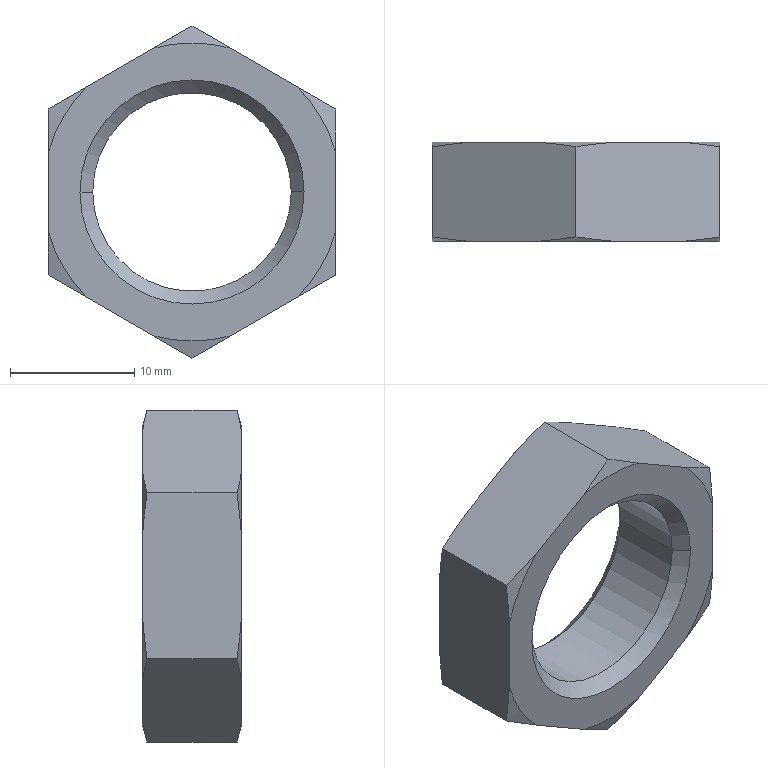Component | SolidWorks | GB_T6172.1-2000HexThinNutAAndBM16-3 | 1 solid | 26 faces | box 23.17 x 8 x 26.75 mm | volume 2049 mm3 | cone 16 | plane 8 | cylinder 2 | commonest cylinder face diameters 16 x2 | material 04 Grade
STEP:
#1=CARTESIAN_POINT('',(-12.126,-0.5893,-13.85));
#2=VERTEX_POINT('',#1);
#3=CARTESIAN_POINT('',(-11.496,-0.5893,-13.847));
#4=VERTEX_POINT('',#3);
#5=CARTESIAN_POINT('',(-11.811,-0.5893,-13.848));
#6=DIRECTION('',(0.,-1.,-0.));
#7=DIRECTION('',(-1.,0.,-0.003934));
#8=AXIS2_PLACEMENT_3D('',#5,#6,#7);
#9=CIRCLE('',#8,0.315);
#10=EDGE_CURVE('',#2,#4,#9,.T.);
#11=ORIENTED_EDGE('',*,*,#10,.F.);
#12=CARTESIAN_POINT('',(-12.167,-0.6299,-13.85));
#13=VERTEX_POINT('',#12);
#14=CARTESIAN_POINT('',(-12.126,-0.5893,-13.85));
#15=DIRECTION('',(-0.7071,-0.7071,-0.002781));
#16=VECTOR('',#15,39.37);
#17=LINE('',#14,#16);
#18=EDGE_CURVE('',#2,#13,#17,.T.);
#19=ORIENTED_EDGE('',*,*,#18,.T.);
#20=CARTESIAN_POINT('',(-11.455,-0.6299,-13.847));
#21=VERTEX_POINT('',#20);
#22=CARTESIAN_POINT('',(-11.811,-0.6299,-13.848));
#23=DIRECTION('',(-0.,1.,0.));
#24=DIRECTION('',(-1.,0.,-0.003934));
#25=AXIS2_PLACEMENT_3D('',#22,#23,#24);
#26=CIRCLE('',#25,0.3555);
#27=EDGE_CURVE('',#21,#13,#26,.T.);
#28=ORIENTED_EDGE('',*,*,#27,.F.);
#29=CARTESIAN_POINT('',(-11.496,-0.5893,-13.847));
#30=DIRECTION('',(0.7071,-0.7071,0.002781));
#31=VECTOR('',#30,39.37);
#32=LINE('',#29,#31);
#33=EDGE_CURVE('',#4,#21,#32,.T.);
#34=ORIENTED_EDGE('',*,*,#33,.F.);
#35=EDGE_LOOP('',(#11,#19,#28,#34));
#36=FACE_OUTER_BOUND('',#35,.T.);
#37=CARTESIAN_POINT('',(-11.811,-0.5893,-13.848));
#38=DIRECTION('',(0.,-1.,-0.));
#39=DIRECTION('',(1.,0.,0.003934));
#40=AXIS2_PLACEMENT_3D('',#37,#38,#39);
#41=CONICAL_SURFACE('',#40,0.315,0.7854);
#42=ADVANCED_FACE('',(#36),#41,.F.);
#43=CARTESIAN_POINT('',(-11.496,-0.3555,-13.847));
#44=VERTEX_POINT('',#43);
#45=CARTESIAN_POINT('',(-12.126,-0.3555,-13.85));
#46=VERTEX_POINT('',#45);
#47=CARTESIAN_POINT('',(-11.811,-0.3555,-13.848));
#48=DIRECTION('',(-0.,1.,0.));
#49=DIRECTION('',(-1.,0.,-0.003934));
#50=AXIS2_PLACEMENT_3D('',#47,#48,#49);
#51=CIRCLE('',#50,0.315);
#52=EDGE_CURVE('',#44,#46,#51,.T.);
#53=ORIENTED_EDGE('',*,*,#52,.F.);
#54=CARTESIAN_POINT('',(-11.455,-0.315,-13.847));
#55=VERTEX_POINT('',#54);
#56=CARTESIAN_POINT('',(-11.455,-0.315,-13.847));
#57=DIRECTION('',(0.7071,0.7071,0.002781));
#58=VECTOR('',#57,39.37);
#59=LINE('',#56,#58);
#60=EDGE_CURVE('',#44,#55,#59,.T.);
#61=ORIENTED_EDGE('',*,*,#60,.T.);
#62=CARTESIAN_POINT('',(-12.167,-0.315,-13.85));
#63=VERTEX_POINT('',#62);
#64=CARTESIAN_POINT('',(-11.811,-0.315,-13.848));
#65=DIRECTION('',(0.,-1.,-0.));
#66=DIRECTION('',(-1.,0.,-0.003934));
#67=AXIS2_PLACEMENT_3D('',#64,#65,#66);
#68=CIRCLE('',#67,0.3555);
#69=EDGE_CURVE('',#63,#55,#68,.T.);
#70=ORIENTED_EDGE('',*,*,#69,.F.);
#71=CARTESIAN_POINT('',(-12.167,-0.315,-13.85));
#72=DIRECTION('',(-0.7071,0.7071,-0.002781));
#73=VECTOR('',#72,39.37);
#74=LINE('',#71,#73);
#75=EDGE_CURVE('',#46,#63,#74,.T.);
#76=ORIENTED_EDGE('',*,*,#75,.F.);
#77=EDGE_LOOP('',(#53,#61,#70,#76));
#78=FACE_OUTER_BOUND('',#77,.T.);
#79=CARTESIAN_POINT('',(-11.811,-0.315,-13.848));
#80=DIRECTION('',(-0.,1.,0.));
#81=DIRECTION('',(-1.,0.,-0.003934));
#82=AXIS2_PLACEMENT_3D('',#79,#80,#81);
#83=CONICAL_SURFACE('',#82,0.3555,0.7854);
#84=ADVANCED_FACE('',(#78),#83,.F.);
#85=ORIENTED_EDGE('',*,*,#10,.T.);
#86=CARTESIAN_POINT('',(-11.496,-0.6299,-13.847));
#87=DIRECTION('',(-0.,1.,0.));
#88=VECTOR('',#87,39.37);
#89=LINE('',#86,#88);
#90=EDGE_CURVE('',#4,#44,#89,.T.);
#91=ORIENTED_EDGE('',*,*,#90,.T.);
#92=ORIENTED_EDGE('',*,*,#52,.T.);
#93=CARTESIAN_POINT('',(-12.126,-0.6299,-13.85));
#94=DIRECTION('',(-0.,1.,0.));
#95=VECTOR('',#94,39.37);
#96=LINE('',#93,#95);
#97=EDGE_CURVE('',#2,#46,#96,.T.);
#98=ORIENTED_EDGE('',*,*,#97,.F.);
#99=EDGE_LOOP('',(#85,#91,#92,#98));
#100=FACE_OUTER_BOUND('',#99,.T.);
#101=CARTESIAN_POINT('',(-11.811,-0.6299,-13.848));
#102=DIRECTION('',(-0.,1.,0.));
#103=DIRECTION('',(-1.,0.,-0.003934));
#104=AXIS2_PLACEMENT_3D('',#101,#102,#103);
#105=CYLINDRICAL_SURFACE('',#104,0.315);
#106=ADVANCED_FACE('',(#100),#105,.F.);
#107=CARTESIAN_POINT('',(-11.355,-0.6154,-13.585));
#108=VERTEX_POINT('',#107);
#109=CARTESIAN_POINT('',(-11.476,-0.6299,-13.515));
#110=VERTEX_POINT('',#109);
#111=CARTESIAN_POINT('',(-11.355,-0.6154,-13.585));
#112=CARTESIAN_POINT('',(-11.395,-0.6216,-13.562));
#113=CARTESIAN_POINT('',(-11.436,-0.6266,-13.539));
#114=CARTESIAN_POINT('',(-11.476,-0.6299,-13.515));
#115=B_SPLINE_CURVE_WITH_KNOTS('',3,(#111,#112,#113,#114),.UNSPECIFIED.,.F.,.F.,(4,4),(0.01098,0.01455),.UNSPECIFIED.);
#116=EDGE_CURVE('',#108,#110,#115,.T.);
#117=ORIENTED_EDGE('',*,*,#116,.F.);
#118=CARTESIAN_POINT('',(-11.355,-0.3295,-13.585));
#119=VERTEX_POINT('',#118);
#120=CARTESIAN_POINT('',(-11.355,-0.6299,-13.585));
#121=DIRECTION('',(-0.,1.,0.));
#122=VECTOR('',#121,39.37);
#123=LINE('',#120,#122);
#124=EDGE_CURVE('',#108,#119,#123,.T.);
#125=ORIENTED_EDGE('',*,*,#124,.T.);
#126=CARTESIAN_POINT('',(-11.476,-0.315,-13.515));
#127=VERTEX_POINT('',#126);
#128=CARTESIAN_POINT('',(-11.476,-0.315,-13.515));
#129=CARTESIAN_POINT('',(-11.456,-0.3166,-13.527));
#130=CARTESIAN_POINT('',(-11.436,-0.3187,-13.539));
#131=CARTESIAN_POINT('',(-11.395,-0.3236,-13.562));
#132=CARTESIAN_POINT('',(-11.375,-0.3264,-13.574));
#133=CARTESIAN_POINT('',(-11.355,-0.3295,-13.585));
#134=B_SPLINE_CURVE_WITH_KNOTS('',3,(#128,#129,#130,#131,#132,#133),.UNSPECIFIED.,.F.,.F.,(4,2,4),(0.02079,0.02254,0.0243),.UNSPECIFIED.);
#135=EDGE_CURVE('',#127,#119,#134,.T.);
#136=ORIENTED_EDGE('',*,*,#135,.F.);
#137=CARTESIAN_POINT('',(-11.69,-0.315,-13.392));
#138=VERTEX_POINT('',#137);
#139=CARTESIAN_POINT('',(-11.355,-0.315,-13.585));
#140=DIRECTION('',(-0.866,-0.,0.5));
#141=VECTOR('',#140,39.37);
#142=LINE('',#139,#141);
#143=EDGE_CURVE('',#127,#138,#142,.T.);
#144=ORIENTED_EDGE('',*,*,#143,.T.);
#145=CARTESIAN_POINT('',(-11.811,-0.3295,-13.322));
#146=VERTEX_POINT('',#145);
#147=CARTESIAN_POINT('',(-11.811,-0.3295,-13.322));
#148=CARTESIAN_POINT('',(-11.771,-0.3232,-13.345));
#149=CARTESIAN_POINT('',(-11.73,-0.3182,-13.368));
#150=CARTESIAN_POINT('',(-11.69,-0.315,-13.392));
#151=B_SPLINE_CURVE_WITH_KNOTS('',3,(#147,#148,#149,#150),.UNSPECIFIED.,.F.,.F.,(4,4),(0.01098,0.01455),.UNSPECIFIED.);
#152=EDGE_CURVE('',#146,#138,#151,.T.);
#153=ORIENTED_EDGE('',*,*,#152,.F.);
#154=CARTESIAN_POINT('',(-11.811,-0.6154,-13.322));
#155=VERTEX_POINT('',#154);
#156=CARTESIAN_POINT('',(-11.811,-0.6299,-13.322));
#157=DIRECTION('',(-0.,1.,0.));
#158=VECTOR('',#157,39.37);
#159=LINE('',#156,#158);
#160=EDGE_CURVE('',#155,#146,#159,.T.);
#161=ORIENTED_EDGE('',*,*,#160,.F.);
#162=CARTESIAN_POINT('',(-11.69,-0.6299,-13.392));
#163=VERTEX_POINT('',#162);
#164=CARTESIAN_POINT('',(-11.69,-0.6299,-13.392));
#165=CARTESIAN_POINT('',(-11.71,-0.6283,-13.38));
#166=CARTESIAN_POINT('',(-11.73,-0.6262,-13.368));
#167=CARTESIAN_POINT('',(-11.771,-0.6213,-13.345));
#168=CARTESIAN_POINT('',(-11.791,-0.6185,-13.333));
#169=CARTESIAN_POINT('',(-11.811,-0.6154,-13.322));
#170=B_SPLINE_CURVE_WITH_KNOTS('',3,(#164,#165,#166,#167,#168,#169),.UNSPECIFIED.,.F.,.F.,(4,2,4),(0.02079,0.02254,0.0243),.UNSPECIFIED.);
#171=EDGE_CURVE('',#163,#155,#170,.T.);
#172=ORIENTED_EDGE('',*,*,#171,.F.);
#173=CARTESIAN_POINT('',(-11.355,-0.6299,-13.585));
#174=DIRECTION('',(-0.866,-0.,0.5));
#175=VECTOR('',#174,39.37);
#176=LINE('',#173,#175);
#177=EDGE_CURVE('',#110,#163,#176,.T.);
#178=ORIENTED_EDGE('',*,*,#177,.F.);
#179=EDGE_LOOP('',(#117,#125,#136,#144,#153,#161,#172,#178));
#180=FACE_OUTER_BOUND('',#179,.T.);
#181=CARTESIAN_POINT('',(-11.355,-0.6299,-13.585));
#182=DIRECTION('',(-0.5,0.,-0.866));
#183=DIRECTION('',(0.866,0.,-0.5));
#184=AXIS2_PLACEMENT_3D('',#181,#182,#183);
#185=PLANE('',#184);
#186=ADVANCED_FACE('',(#180),#185,.F.);
#187=CARTESIAN_POINT('',(-11.932,-0.6299,-13.392));
#188=VERTEX_POINT('',#187);
#189=CARTESIAN_POINT('',(-11.811,-0.6154,-13.322));
#190=CARTESIAN_POINT('',(-11.851,-0.6216,-13.345));
#191=CARTESIAN_POINT('',(-11.892,-0.6266,-13.368));
#192=CARTESIAN_POINT('',(-11.932,-0.6299,-13.392));
#193=B_SPLINE_CURVE_WITH_KNOTS('',3,(#189,#190,#191,#192),.UNSPECIFIED.,.F.,.F.,(4,4),(0.01093,0.0145),.UNSPECIFIED.);
#194=EDGE_CURVE('',#155,#188,#193,.T.);
#195=ORIENTED_EDGE('',*,*,#194,.F.);
#196=ORIENTED_EDGE('',*,*,#160,.T.);
#197=CARTESIAN_POINT('',(-11.932,-0.315,-13.392));
#198=VERTEX_POINT('',#197);
#199=CARTESIAN_POINT('',(-11.932,-0.315,-13.392));
#200=CARTESIAN_POINT('',(-11.912,-0.3166,-13.38));
#201=CARTESIAN_POINT('',(-11.892,-0.3187,-13.368));
#202=CARTESIAN_POINT('',(-11.851,-0.3236,-13.345));
#203=CARTESIAN_POINT('',(-11.831,-0.3264,-13.333));
#204=CARTESIAN_POINT('',(-11.811,-0.3295,-13.322));
#205=B_SPLINE_CURVE_WITH_KNOTS('',3,(#199,#200,#201,#202,#203,#204),.UNSPECIFIED.,.F.,.F.,(4,2,4),(0.02074,0.02249,0.02425),.UNSPECIFIED.);
#206=EDGE_CURVE('',#198,#146,#205,.T.);
#207=ORIENTED_EDGE('',*,*,#206,.F.);
#208=CARTESIAN_POINT('',(-12.146,-0.315,-13.515));
#209=VERTEX_POINT('',#208);
#210=CARTESIAN_POINT('',(-11.811,-0.315,-13.322));
#211=DIRECTION('',(-0.866,0.,-0.5));
#212=VECTOR('',#211,39.37);
#213=LINE('',#210,#212);
#214=EDGE_CURVE('',#198,#209,#213,.T.);
#215=ORIENTED_EDGE('',*,*,#214,.T.);
#216=CARTESIAN_POINT('',(-12.267,-0.3295,-13.585));
#217=VERTEX_POINT('',#216);
#218=CARTESIAN_POINT('',(-12.267,-0.3295,-13.585));
#219=CARTESIAN_POINT('',(-12.227,-0.3232,-13.562));
#220=CARTESIAN_POINT('',(-12.186,-0.3182,-13.539));
#221=CARTESIAN_POINT('',(-12.146,-0.315,-13.515));
#222=B_SPLINE_CURVE_WITH_KNOTS('',3,(#218,#219,#220,#221),.UNSPECIFIED.,.F.,.F.,(4,4),(0.01093,0.0145),.UNSPECIFIED.);
#223=EDGE_CURVE('',#217,#209,#222,.T.);
#224=ORIENTED_EDGE('',*,*,#223,.F.);
#225=CARTESIAN_POINT('',(-12.267,-0.6154,-13.585));
#226=VERTEX_POINT('',#225);
#227=CARTESIAN_POINT('',(-12.267,-0.6299,-13.585));
#228=DIRECTION('',(-0.,1.,0.));
#229=VECTOR('',#228,39.37);
#230=LINE('',#227,#229);
#231=EDGE_CURVE('',#226,#217,#230,.T.);
#232=ORIENTED_EDGE('',*,*,#231,.F.);
#233=CARTESIAN_POINT('',(-12.146,-0.6299,-13.515));
#234=VERTEX_POINT('',#233);
#235=CARTESIAN_POINT('',(-12.146,-0.6299,-13.515));
#236=CARTESIAN_POINT('',(-12.166,-0.6283,-13.527));
#237=CARTESIAN_POINT('',(-12.186,-0.6262,-13.539));
#238=CARTESIAN_POINT('',(-12.227,-0.6213,-13.562));
#239=CARTESIAN_POINT('',(-12.247,-0.6185,-13.574));
#240=CARTESIAN_POINT('',(-12.267,-0.6154,-13.585));
#241=B_SPLINE_CURVE_WITH_KNOTS('',3,(#235,#236,#237,#238,#239,#240),.UNSPECIFIED.,.F.,.F.,(4,2,4),(0.02074,0.02249,0.02425),.UNSPECIFIED.);
#242=EDGE_CURVE('',#234,#226,#241,.T.);
#243=ORIENTED_EDGE('',*,*,#242,.F.);
#244=CARTESIAN_POINT('',(-11.811,-0.6299,-13.322));
#245=DIRECTION('',(-0.866,0.,-0.5));
#246=VECTOR('',#245,39.37);
#247=LINE('',#244,#246);
#248=EDGE_CURVE('',#188,#234,#247,.T.);
#249=ORIENTED_EDGE('',*,*,#248,.F.);
#250=EDGE_LOOP('',(#195,#196,#207,#215,#224,#232,#243,#249));
#251=FACE_OUTER_BOUND('',#250,.T.);
#252=CARTESIAN_POINT('',(-11.811,-0.6299,-13.322));
#253=DIRECTION('',(0.5,0.,-0.866));
#254=DIRECTION('',(0.866,-0.,0.5));
#255=AXIS2_PLACEMENT_3D('',#252,#253,#254);
#256=PLANE('',#255);
#257=ADVANCED_FACE('',(#251),#256,.F.);
#258=CARTESIAN_POINT('',(-12.267,-0.6299,-13.725));
#259=VERTEX_POINT('',#258);
#260=CARTESIAN_POINT('',(-12.267,-0.6154,-13.585));
#261=CARTESIAN_POINT('',(-12.267,-0.6216,-13.632));
#262=CARTESIAN_POINT('',(-12.267,-0.6266,-13.678));
#263=CARTESIAN_POINT('',(-12.267,-0.6299,-13.725));
#264=B_SPLINE_CURVE_WITH_KNOTS('',3,(#260,#261,#262,#263),.UNSPECIFIED.,.F.,.F.,(4,4),(0.009475,0.01305),.UNSPECIFIED.);
#265=EDGE_CURVE('',#226,#259,#264,.T.);
#266=ORIENTED_EDGE('',*,*,#265,.F.);
#267=ORIENTED_EDGE('',*,*,#231,.T.);
#268=CARTESIAN_POINT('',(-12.267,-0.315,-13.725));
#269=VERTEX_POINT('',#268);
#270=CARTESIAN_POINT('',(-12.267,-0.315,-13.725));
#271=CARTESIAN_POINT('',(-12.267,-0.3166,-13.702));
#272=CARTESIAN_POINT('',(-12.267,-0.3187,-13.678));
#273=CARTESIAN_POINT('',(-12.267,-0.3235,-13.632));
#274=CARTESIAN_POINT('',(-12.267,-0.3264,-13.608));
#275=CARTESIAN_POINT('',(-12.267,-0.3295,-13.585));
#276=B_SPLINE_CURVE_WITH_KNOTS('',3,(#270,#271,#272,#273,#274,#275),.UNSPECIFIED.,.F.,.F.,(4,2,4),(0.01929,0.02104,0.0228),.UNSPECIFIED.);
#277=EDGE_CURVE('',#269,#217,#276,.T.);
#278=ORIENTED_EDGE('',*,*,#277,.F.);
#279=CARTESIAN_POINT('',(-12.267,-0.315,-13.972));
#280=VERTEX_POINT('',#279);
#281=CARTESIAN_POINT('',(-12.267,-0.315,-13.585));
#282=DIRECTION('',(-0.,0.,-1.));
#283=VECTOR('',#282,39.37);
#284=LINE('',#281,#283);
#285=EDGE_CURVE('',#269,#280,#284,.T.);
#286=ORIENTED_EDGE('',*,*,#285,.T.);
#287=CARTESIAN_POINT('',(-12.267,-0.3295,-14.112));
#288=VERTEX_POINT('',#287);
#289=CARTESIAN_POINT('',(-12.267,-0.3295,-14.112));
#290=CARTESIAN_POINT('',(-12.267,-0.3232,-14.065));
#291=CARTESIAN_POINT('',(-12.267,-0.3182,-14.019));
#292=CARTESIAN_POINT('',(-12.267,-0.315,-13.972));
#293=B_SPLINE_CURVE_WITH_KNOTS('',3,(#289,#290,#291,#292),.UNSPECIFIED.,.F.,.F.,(4,4),(0.009475,0.01305),.UNSPECIFIED.);
#294=EDGE_CURVE('',#288,#280,#293,.T.);
#295=ORIENTED_EDGE('',*,*,#294,.F.);
#296=CARTESIAN_POINT('',(-12.267,-0.6154,-14.112));
#297=VERTEX_POINT('',#296);
#298=CARTESIAN_POINT('',(-12.267,-0.6299,-14.112));
#299=DIRECTION('',(-0.,1.,0.));
#300=VECTOR('',#299,39.37);
#301=LINE('',#298,#300);
#302=EDGE_CURVE('',#297,#288,#301,.T.);
#303=ORIENTED_EDGE('',*,*,#302,.F.);
#304=CARTESIAN_POINT('',(-12.267,-0.6299,-13.972));
#305=VERTEX_POINT('',#304);
#306=CARTESIAN_POINT('',(-12.267,-0.6299,-13.972));
#307=CARTESIAN_POINT('',(-12.267,-0.6283,-13.995));
#308=CARTESIAN_POINT('',(-12.267,-0.6262,-14.019));
#309=CARTESIAN_POINT('',(-12.267,-0.6213,-14.065));
#310=CARTESIAN_POINT('',(-12.267,-0.6185,-14.089));
#311=CARTESIAN_POINT('',(-12.267,-0.6154,-14.112));
#312=B_SPLINE_CURVE_WITH_KNOTS('',3,(#306,#307,#308,#309,#310,#311),.UNSPECIFIED.,.F.,.F.,(4,2,4),(0.01929,0.02104,0.0228),.UNSPECIFIED.);
#313=EDGE_CURVE('',#305,#297,#312,.T.);
#314=ORIENTED_EDGE('',*,*,#313,.F.);
#315=CARTESIAN_POINT('',(-12.267,-0.6299,-13.585));
#316=DIRECTION('',(-0.,0.,-1.));
#317=VECTOR('',#316,39.37);
#318=LINE('',#315,#317);
#319=EDGE_CURVE('',#259,#305,#318,.T.);
#320=ORIENTED_EDGE('',*,*,#319,.F.);
#321=EDGE_LOOP('',(#266,#267,#278,#286,#295,#303,#314,#320));
#322=FACE_OUTER_BOUND('',#321,.T.);
#323=CARTESIAN_POINT('',(-12.267,-0.6299,-13.585));
#324=DIRECTION('',(1.,0.,-0.));
#325=DIRECTION('',(0.,-0.,1.));
#326=AXIS2_PLACEMENT_3D('',#323,#324,#325);
#327=PLANE('',#326);
#328=ADVANCED_FACE('',(#322),#327,.F.);
#329=CARTESIAN_POINT('',(-12.146,-0.6299,-14.182));
#330=VERTEX_POINT('',#329);
#331=CARTESIAN_POINT('',(-12.267,-0.6154,-14.112));
#332=CARTESIAN_POINT('',(-12.227,-0.6216,-14.135));
#333=CARTESIAN_POINT('',(-12.186,-0.6266,-14.158));
#334=CARTESIAN_POINT('',(-12.146,-0.6299,-14.182));
#335=B_SPLINE_CURVE_WITH_KNOTS('',3,(#331,#332,#333,#334),.UNSPECIFIED.,.F.,.F.,(4,4),(0.01098,0.01455),.UNSPECIFIED.);
#336=EDGE_CURVE('',#297,#330,#335,.T.);
#337=ORIENTED_EDGE('',*,*,#336,.F.);
#338=ORIENTED_EDGE('',*,*,#302,.T.);
#339=CARTESIAN_POINT('',(-12.146,-0.315,-14.182));
#340=VERTEX_POINT('',#339);
#341=CARTESIAN_POINT('',(-12.146,-0.315,-14.182));
#342=CARTESIAN_POINT('',(-12.166,-0.3166,-14.17));
#343=CARTESIAN_POINT('',(-12.186,-0.3187,-14.158));
#344=CARTESIAN_POINT('',(-12.227,-0.3236,-14.135));
#345=CARTESIAN_POINT('',(-12.247,-0.3264,-14.123));
#346=CARTESIAN_POINT('',(-12.267,-0.3295,-14.112));
#347=B_SPLINE_CURVE_WITH_KNOTS('',3,(#341,#342,#343,#344,#345,#346),.UNSPECIFIED.,.F.,.F.,(4,2,4),(0.02079,0.02254,0.0243),.UNSPECIFIED.);
#348=EDGE_CURVE('',#340,#288,#347,.T.);
#349=ORIENTED_EDGE('',*,*,#348,.F.);
#350=CARTESIAN_POINT('',(-11.932,-0.315,-14.305));
#351=VERTEX_POINT('',#350);
#352=CARTESIAN_POINT('',(-12.267,-0.315,-14.112));
#353=DIRECTION('',(0.866,0.,-0.5));
#354=VECTOR('',#353,39.37);
#355=LINE('',#352,#354);
#356=EDGE_CURVE('',#340,#351,#355,.T.);
#357=ORIENTED_EDGE('',*,*,#356,.T.);
#358=CARTESIAN_POINT('',(-11.811,-0.3295,-14.375));
#359=VERTEX_POINT('',#358);
#360=CARTESIAN_POINT('',(-11.811,-0.3295,-14.375));
#361=CARTESIAN_POINT('',(-11.851,-0.3232,-14.352));
#362=CARTESIAN_POINT('',(-11.892,-0.3182,-14.328));
#363=CARTESIAN_POINT('',(-11.932,-0.315,-14.305));
#364=B_SPLINE_CURVE_WITH_KNOTS('',3,(#360,#361,#362,#363),.UNSPECIFIED.,.F.,.F.,(4,4),(0.01098,0.01455),.UNSPECIFIED.);
#365=EDGE_CURVE('',#359,#351,#364,.T.);
#366=ORIENTED_EDGE('',*,*,#365,.F.);
#367=CARTESIAN_POINT('',(-11.811,-0.6154,-14.375));
#368=VERTEX_POINT('',#367);
#369=CARTESIAN_POINT('',(-11.811,-0.6299,-14.375));
#370=DIRECTION('',(-0.,1.,0.));
#371=VECTOR('',#370,39.37);
#372=LINE('',#369,#371);
#373=EDGE_CURVE('',#368,#359,#372,.T.);
#374=ORIENTED_EDGE('',*,*,#373,.F.);
#375=CARTESIAN_POINT('',(-11.932,-0.6299,-14.305));
#376=VERTEX_POINT('',#375);
#377=CARTESIAN_POINT('',(-11.932,-0.6299,-14.305));
#378=CARTESIAN_POINT('',(-11.912,-0.6283,-14.317));
#379=CARTESIAN_POINT('',(-11.892,-0.6262,-14.328));
#380=CARTESIAN_POINT('',(-11.851,-0.6213,-14.352));
#381=CARTESIAN_POINT('',(-11.831,-0.6185,-14.363));
#382=CARTESIAN_POINT('',(-11.811,-0.6154,-14.375));
#383=B_SPLINE_CURVE_WITH_KNOTS('',3,(#377,#378,#379,#380,#381,#382),.UNSPECIFIED.,.F.,.F.,(4,2,4),(0.02079,0.02254,0.0243),.UNSPECIFIED.);
#384=EDGE_CURVE('',#376,#368,#383,.T.);
#385=ORIENTED_EDGE('',*,*,#384,.F.);
#386=CARTESIAN_POINT('',(-12.267,-0.6299,-14.112));
#387=DIRECTION('',(0.866,0.,-0.5));
#388=VECTOR('',#387,39.37);
#389=LINE('',#386,#388);
#390=EDGE_CURVE('',#330,#376,#389,.T.);
#391=ORIENTED_EDGE('',*,*,#390,.F.);
#392=EDGE_LOOP('',(#337,#338,#349,#357,#366,#374,#385,#391));
#393=FACE_OUTER_BOUND('',#392,.T.);
#394=CARTESIAN_POINT('',(-12.267,-0.6299,-14.112));
#395=DIRECTION('',(0.5,-0.,0.866));
#396=DIRECTION('',(-0.866,-0.,0.5));
#397=AXIS2_PLACEMENT_3D('',#394,#395,#396);
#398=PLANE('',#397);
#399=ADVANCED_FACE('',(#393),#398,.F.);
#400=CARTESIAN_POINT('',(-11.69,-0.6299,-14.305));
#401=VERTEX_POINT('',#400);
#402=CARTESIAN_POINT('',(-11.811,-0.6154,-14.375));
#403=CARTESIAN_POINT('',(-11.771,-0.6216,-14.352));
#404=CARTESIAN_POINT('',(-11.73,-0.6266,-14.328));
#405=CARTESIAN_POINT('',(-11.69,-0.6299,-14.305));
#406=B_SPLINE_CURVE_WITH_KNOTS('',3,(#402,#403,#404,#405),.UNSPECIFIED.,.F.,.F.,(4,4),(0.01093,0.0145),.UNSPECIFIED.);
#407=EDGE_CURVE('',#368,#401,#406,.T.);
#408=ORIENTED_EDGE('',*,*,#407,.F.);
#409=ORIENTED_EDGE('',*,*,#373,.T.);
#410=CARTESIAN_POINT('',(-11.69,-0.315,-14.305));
#411=VERTEX_POINT('',#410);
#412=CARTESIAN_POINT('',(-11.69,-0.315,-14.305));
#413=CARTESIAN_POINT('',(-11.71,-0.3166,-14.317));
#414=CARTESIAN_POINT('',(-11.73,-0.3187,-14.328));
#415=CARTESIAN_POINT('',(-11.771,-0.3236,-14.352));
#416=CARTESIAN_POINT('',(-11.791,-0.3264,-14.363));
#417=CARTESIAN_POINT('',(-11.811,-0.3295,-14.375));
#418=B_SPLINE_CURVE_WITH_KNOTS('',3,(#412,#413,#414,#415,#416,#417),.UNSPECIFIED.,.F.,.F.,(4,2,4),(0.02074,0.02249,0.02425),.UNSPECIFIED.);
#419=EDGE_CURVE('',#411,#359,#418,.T.);
#420=ORIENTED_EDGE('',*,*,#419,.F.);
#421=CARTESIAN_POINT('',(-11.476,-0.315,-14.182));
#422=VERTEX_POINT('',#421);
#423=CARTESIAN_POINT('',(-11.811,-0.315,-14.375));
#424=DIRECTION('',(0.866,-0.,0.5));
#425=VECTOR('',#424,39.37);
#426=LINE('',#423,#425);
#427=EDGE_CURVE('',#411,#422,#426,.T.);
#428=ORIENTED_EDGE('',*,*,#427,.T.);
#429=CARTESIAN_POINT('',(-11.355,-0.3295,-14.112));
#430=VERTEX_POINT('',#429);
#431=CARTESIAN_POINT('',(-11.355,-0.3295,-14.112));
#432=CARTESIAN_POINT('',(-11.395,-0.3232,-14.135));
#433=CARTESIAN_POINT('',(-11.436,-0.3182,-14.158));
#434=CARTESIAN_POINT('',(-11.476,-0.315,-14.182));
#435=B_SPLINE_CURVE_WITH_KNOTS('',3,(#431,#432,#433,#434),.UNSPECIFIED.,.F.,.F.,(4,4),(0.01093,0.0145),.UNSPECIFIED.);
#436=EDGE_CURVE('',#430,#422,#435,.T.);
#437=ORIENTED_EDGE('',*,*,#436,.F.);
#438=CARTESIAN_POINT('',(-11.355,-0.6154,-14.112));
#439=VERTEX_POINT('',#438);
#440=CARTESIAN_POINT('',(-11.355,-0.6299,-14.112));
#441=DIRECTION('',(-0.,1.,0.));
#442=VECTOR('',#441,39.37);
#443=LINE('',#440,#442);
#444=EDGE_CURVE('',#439,#430,#443,.T.);
#445=ORIENTED_EDGE('',*,*,#444,.F.);
#446=CARTESIAN_POINT('',(-11.476,-0.6299,-14.182));
#447=VERTEX_POINT('',#446);
#448=CARTESIAN_POINT('',(-11.476,-0.6299,-14.182));
#449=CARTESIAN_POINT('',(-11.456,-0.6283,-14.17));
#450=CARTESIAN_POINT('',(-11.436,-0.6262,-14.158));
#451=CARTESIAN_POINT('',(-11.395,-0.6213,-14.135));
#452=CARTESIAN_POINT('',(-11.375,-0.6185,-14.123));
#453=CARTESIAN_POINT('',(-11.355,-0.6154,-14.112));
#454=B_SPLINE_CURVE_WITH_KNOTS('',3,(#448,#449,#450,#451,#452,#453),.UNSPECIFIED.,.F.,.F.,(4,2,4),(0.02074,0.02249,0.02425),.UNSPECIFIED.);
#455=EDGE_CURVE('',#447,#439,#454,.T.);
#456=ORIENTED_EDGE('',*,*,#455,.F.);
#457=CARTESIAN_POINT('',(-11.811,-0.6299,-14.375));
#458=DIRECTION('',(0.866,-0.,0.5));
#459=VECTOR('',#458,39.37);
#460=LINE('',#457,#459);
#461=EDGE_CURVE('',#401,#447,#460,.T.);
#462=ORIENTED_EDGE('',*,*,#461,.F.);
#463=EDGE_LOOP('',(#408,#409,#420,#428,#437,#445,#456,#462));
#464=FACE_OUTER_BOUND('',#463,.T.);
#465=CARTESIAN_POINT('',(-11.811,-0.6299,-14.375));
#466=DIRECTION('',(-0.5,-0.,0.866));
#467=DIRECTION('',(-0.866,0.,-0.5));
#468=AXIS2_PLACEMENT_3D('',#465,#466,#467);
#469=PLANE('',#468);
#470=ADVANCED_FACE('',(#464),#469,.F.);
#471=CARTESIAN_POINT('',(-11.355,-0.6299,-13.972));
#472=VERTEX_POINT('',#471);
#473=CARTESIAN_POINT('',(-11.355,-0.6154,-14.112));
#474=CARTESIAN_POINT('',(-11.355,-0.6216,-14.065));
#475=CARTESIAN_POINT('',(-11.355,-0.6266,-14.019));
#476=CARTESIAN_POINT('',(-11.355,-0.6299,-13.972));
#477=B_SPLINE_CURVE_WITH_KNOTS('',3,(#473,#474,#475,#476),.UNSPECIFIED.,.F.,.F.,(4,4),(0.009475,0.01305),.UNSPECIFIED.);
#478=EDGE_CURVE('',#439,#472,#477,.T.);
#479=ORIENTED_EDGE('',*,*,#478,.F.);
#480=ORIENTED_EDGE('',*,*,#444,.T.);
#481=CARTESIAN_POINT('',(-11.355,-0.315,-13.972));
#482=VERTEX_POINT('',#481);
#483=CARTESIAN_POINT('',(-11.355,-0.315,-13.972));
#484=CARTESIAN_POINT('',(-11.355,-0.3166,-13.995));
#485=CARTESIAN_POINT('',(-11.355,-0.3187,-14.019));
#486=CARTESIAN_POINT('',(-11.355,-0.3235,-14.065));
#487=CARTESIAN_POINT('',(-11.355,-0.3264,-14.089));
#488=CARTESIAN_POINT('',(-11.355,-0.3295,-14.112));
#489=B_SPLINE_CURVE_WITH_KNOTS('',3,(#483,#484,#485,#486,#487,#488),.UNSPECIFIED.,.F.,.F.,(4,2,4),(0.01929,0.02104,0.0228),.UNSPECIFIED.);
#490=EDGE_CURVE('',#482,#430,#489,.T.);
#491=ORIENTED_EDGE('',*,*,#490,.F.);
#492=CARTESIAN_POINT('',(-11.355,-0.315,-13.725));
#493=VERTEX_POINT('',#492);
#494=CARTESIAN_POINT('',(-11.355,-0.315,-14.112));
#495=DIRECTION('',(0.,-0.,1.));
#496=VECTOR('',#495,39.37);
#497=LINE('',#494,#496);
#498=EDGE_CURVE('',#482,#493,#497,.T.);
#499=ORIENTED_EDGE('',*,*,#498,.T.);
#500=CARTESIAN_POINT('',(-11.355,-0.3295,-13.585));
#501=CARTESIAN_POINT('',(-11.355,-0.3232,-13.632));
#502=CARTESIAN_POINT('',(-11.355,-0.3182,-13.678));
#503=CARTESIAN_POINT('',(-11.355,-0.315,-13.725));
#504=B_SPLINE_CURVE_WITH_KNOTS('',3,(#500,#501,#502,#503),.UNSPECIFIED.,.F.,.F.,(4,4),(0.009475,0.01305),.UNSPECIFIED.);
#505=EDGE_CURVE('',#119,#493,#504,.T.);
#506=ORIENTED_EDGE('',*,*,#505,.F.);
#507=ORIENTED_EDGE('',*,*,#124,.F.);
#508=CARTESIAN_POINT('',(-11.355,-0.6299,-13.725));
#509=VERTEX_POINT('',#508);
#510=CARTESIAN_POINT('',(-11.355,-0.6299,-13.725));
#511=CARTESIAN_POINT('',(-11.355,-0.6283,-13.702));
#512=CARTESIAN_POINT('',(-11.355,-0.6262,-13.678));
#513=CARTESIAN_POINT('',(-11.355,-0.6213,-13.632));
#514=CARTESIAN_POINT('',(-11.355,-0.6185,-13.608));
#515=CARTESIAN_POINT('',(-11.355,-0.6154,-13.585));
#516=B_SPLINE_CURVE_WITH_KNOTS('',3,(#510,#511,#512,#513,#514,#515),.UNSPECIFIED.,.F.,.F.,(4,2,4),(0.01929,0.02104,0.0228),.UNSPECIFIED.);
#517=EDGE_CURVE('',#509,#108,#516,.T.);
#518=ORIENTED_EDGE('',*,*,#517,.F.);
#519=CARTESIAN_POINT('',(-11.355,-0.6299,-14.112));
#520=DIRECTION('',(0.,-0.,1.));
#521=VECTOR('',#520,39.37);
#522=LINE('',#519,#521);
#523=EDGE_CURVE('',#472,#509,#522,.T.);
#524=ORIENTED_EDGE('',*,*,#523,.F.);
#525=EDGE_LOOP('',(#479,#480,#491,#499,#506,#507,#518,#524));
#526=FACE_OUTER_BOUND('',#525,.T.);
#527=CARTESIAN_POINT('',(-11.355,-0.6299,-14.112));
#528=DIRECTION('',(-1.,-0.,0.));
#529=DIRECTION('',(-0.,0.,-1.));
#530=AXIS2_PLACEMENT_3D('',#527,#528,#529);
#531=PLANE('',#530);
#532=ADVANCED_FACE('',(#526),#531,.F.);
#533=ORIENTED_EDGE('',*,*,#27,.T.);
#534=CARTESIAN_POINT('',(-11.811,-0.6299,-13.848));
#535=DIRECTION('',(-0.,1.,0.));
#536=DIRECTION('',(-1.,0.,-0.003934));
#537=AXIS2_PLACEMENT_3D('',#534,#535,#536);
#538=CIRCLE('',#537,0.3555);
#539=EDGE_CURVE('',#13,#21,#538,.T.);
#540=ORIENTED_EDGE('',*,*,#539,.T.);
#541=EDGE_LOOP('',(#533,#540));
#542=FACE_BOUND('',#541,.T.);
#543=CARTESIAN_POINT('',(-11.811,-0.6299,-13.848));
#544=DIRECTION('',(-0.,1.,0.));
#545=DIRECTION('',(-1.,0.,-0.003934));
#546=AXIS2_PLACEMENT_3D('',#543,#544,#545);
#547=CIRCLE('',#546,0.4724);
#548=EDGE_CURVE('',#259,#234,#547,.T.);
#549=ORIENTED_EDGE('',*,*,#548,.F.);
#550=ORIENTED_EDGE('',*,*,#319,.T.);
#551=CARTESIAN_POINT('',(-11.811,-0.6299,-13.848));
#552=DIRECTION('',(-0.,1.,0.));
#553=DIRECTION('',(-1.,0.,-0.003934));
#554=AXIS2_PLACEMENT_3D('',#551,#552,#553);
#555=CIRCLE('',#554,0.4724);
#556=EDGE_CURVE('',#330,#305,#555,.T.);
#557=ORIENTED_EDGE('',*,*,#556,.F.);
#558=ORIENTED_EDGE('',*,*,#390,.T.);
#559=CARTESIAN_POINT('',(-11.811,-0.6299,-13.848));
#560=DIRECTION('',(-0.,1.,0.));
#561=DIRECTION('',(-1.,0.,-0.003934));
#562=AXIS2_PLACEMENT_3D('',#559,#560,#561);
#563=CIRCLE('',#562,0.4724);
#564=EDGE_CURVE('',#401,#376,#563,.T.);
#565=ORIENTED_EDGE('',*,*,#564,.F.);
#566=ORIENTED_EDGE('',*,*,#461,.T.);
#567=CARTESIAN_POINT('',(-11.811,-0.6299,-13.848));
#568=DIRECTION('',(-0.,1.,0.));
#569=DIRECTION('',(-1.,0.,-0.003934));
#570=AXIS2_PLACEMENT_3D('',#567,#568,#569);
#571=CIRCLE('',#570,0.4724);
#572=EDGE_CURVE('',#472,#447,#571,.T.);
#573=ORIENTED_EDGE('',*,*,#572,.F.);
#574=ORIENTED_EDGE('',*,*,#523,.T.);
#575=CARTESIAN_POINT('',(-11.811,-0.6299,-13.848));
#576=DIRECTION('',(0.,-1.,-0.));
#577=DIRECTION('',(1.,0.,0.003934));
#578=AXIS2_PLACEMENT_3D('',#575,#576,#577);
#579=CIRCLE('',#578,0.4724);
#580=EDGE_CURVE('',#509,#110,#579,.T.);
#581=ORIENTED_EDGE('',*,*,#580,.T.);
#582=ORIENTED_EDGE('',*,*,#177,.T.);
#583=CARTESIAN_POINT('',(-11.811,-0.6299,-13.848));
#584=DIRECTION('',(-0.,1.,0.));
#585=DIRECTION('',(-1.,0.,-0.003934));
#586=AXIS2_PLACEMENT_3D('',#583,#584,#585);
#587=CIRCLE('',#586,0.4724);
#588=EDGE_CURVE('',#188,#163,#587,.T.);
#589=ORIENTED_EDGE('',*,*,#588,.F.);
#590=ORIENTED_EDGE('',*,*,#248,.T.);
#591=EDGE_LOOP('',(#549,#550,#557,#558,#565,#566,#573,#574,#581,#582,#589,#590));
#592=FACE_OUTER_BOUND('',#591,.T.);
#593=CARTESIAN_POINT('',(-10.899,-0.6299,-13.848));
#594=DIRECTION('',(-0.,1.,0.));
#595=DIRECTION('',(-1.,-0.,-0.003934));
#596=AXIS2_PLACEMENT_3D('',#593,#594,#595);
#597=PLANE('',#596);
#598=ADVANCED_FACE('',(#542,#592),#597,.F.);
#599=ORIENTED_EDGE('',*,*,#69,.T.);
#600=CARTESIAN_POINT('',(-11.811,-0.315,-13.848));
#601=DIRECTION('',(0.,-1.,-0.));
#602=DIRECTION('',(-1.,0.,-0.003934));
#603=AXIS2_PLACEMENT_3D('',#600,#601,#602);
#604=CIRCLE('',#603,0.3555);
#605=EDGE_CURVE('',#55,#63,#604,.T.);
#606=ORIENTED_EDGE('',*,*,#605,.T.);
#607=EDGE_LOOP('',(#599,#606));
#608=FACE_BOUND('',#607,.T.);
#609=ORIENTED_EDGE('',*,*,#285,.F.);
#610=CARTESIAN_POINT('',(-11.811,-0.315,-13.848));
#611=DIRECTION('',(-0.,1.,0.));
#612=DIRECTION('',(-1.,0.,-0.003934));
#613=AXIS2_PLACEMENT_3D('',#610,#611,#612);
#614=CIRCLE('',#613,0.4724);
#615=EDGE_CURVE('',#269,#209,#614,.T.);
#616=ORIENTED_EDGE('',*,*,#615,.T.);
#617=ORIENTED_EDGE('',*,*,#214,.F.);
#618=CARTESIAN_POINT('',(-11.811,-0.315,-13.848));
#619=DIRECTION('',(-0.,1.,0.));
#620=DIRECTION('',(-1.,0.,-0.003934));
#621=AXIS2_PLACEMENT_3D('',#618,#619,#620);
#622=CIRCLE('',#621,0.4724);
#623=EDGE_CURVE('',#198,#138,#622,.T.);
#624=ORIENTED_EDGE('',*,*,#623,.T.);
#625=ORIENTED_EDGE('',*,*,#143,.F.);
#626=CARTESIAN_POINT('',(-11.811,-0.315,-13.848));
#627=DIRECTION('',(-0.,1.,0.));
#628=DIRECTION('',(-1.,0.,-0.003934));
#629=AXIS2_PLACEMENT_3D('',#626,#627,#628);
#630=CIRCLE('',#629,0.4724);
#631=EDGE_CURVE('',#127,#493,#630,.T.);
#632=ORIENTED_EDGE('',*,*,#631,.T.);
#633=ORIENTED_EDGE('',*,*,#498,.F.);
#634=CARTESIAN_POINT('',(-11.811,-0.315,-13.848));
#635=DIRECTION('',(-0.,1.,0.));
#636=DIRECTION('',(-1.,0.,-0.003934));
#637=AXIS2_PLACEMENT_3D('',#634,#635,#636);
#638=CIRCLE('',#637,0.4724);
#639=EDGE_CURVE('',#482,#422,#638,.T.);
#640=ORIENTED_EDGE('',*,*,#639,.T.);
#641=ORIENTED_EDGE('',*,*,#427,.F.);
#642=CARTESIAN_POINT('',(-11.811,-0.315,-13.848));
#643=DIRECTION('',(-0.,1.,0.));
#644=DIRECTION('',(-1.,0.,-0.003934));
#645=AXIS2_PLACEMENT_3D('',#642,#643,#644);
#646=CIRCLE('',#645,0.4724);
#647=EDGE_CURVE('',#411,#351,#646,.T.);
#648=ORIENTED_EDGE('',*,*,#647,.T.);
#649=ORIENTED_EDGE('',*,*,#356,.F.);
#650=CARTESIAN_POINT('',(-11.811,-0.315,-13.848));
#651=DIRECTION('',(-0.,1.,0.));
#652=DIRECTION('',(-1.,0.,-0.003934));
#653=AXIS2_PLACEMENT_3D('',#650,#651,#652);
#654=CIRCLE('',#653,0.4724);
#655=EDGE_CURVE('',#340,#280,#654,.T.);
#656=ORIENTED_EDGE('',*,*,#655,.T.);
#657=EDGE_LOOP('',(#609,#616,#617,#624,#625,#632,#633,#640,#641,#648,#649,#656));
#658=FACE_OUTER_BOUND('',#657,.T.);
#659=CARTESIAN_POINT('',(-10.899,-0.315,-13.848));
#660=DIRECTION('',(-0.,1.,0.));
#661=DIRECTION('',(-1.,-0.,-0.003934));
#662=AXIS2_PLACEMENT_3D('',#659,#660,#661);
#663=PLANE('',#662);
#664=ADVANCED_FACE('',(#608,#658),#663,.T.);
#665=ORIENTED_EDGE('',*,*,#90,.F.);
#666=CARTESIAN_POINT('',(-11.811,-0.5893,-13.848));
#667=DIRECTION('',(0.,-1.,-0.));
#668=DIRECTION('',(-1.,0.,-0.003934));
#669=AXIS2_PLACEMENT_3D('',#666,#667,#668);
#670=CIRCLE('',#669,0.315);
#671=EDGE_CURVE('',#4,#2,#670,.T.);
#672=ORIENTED_EDGE('',*,*,#671,.T.);
#673=ORIENTED_EDGE('',*,*,#97,.T.);
#674=CARTESIAN_POINT('',(-11.811,-0.3555,-13.848));
#675=DIRECTION('',(-0.,1.,0.));
#676=DIRECTION('',(-1.,0.,-0.003934));
#677=AXIS2_PLACEMENT_3D('',#674,#675,#676);
#678=CIRCLE('',#677,0.315);
#679=EDGE_CURVE('',#46,#44,#678,.T.);
#680=ORIENTED_EDGE('',*,*,#679,.T.);
#681=EDGE_LOOP('',(#665,#672,#673,#680));
#682=FACE_OUTER_BOUND('',#681,.T.);
#683=CARTESIAN_POINT('',(-11.811,-0.6299,-13.848));
#684=DIRECTION('',(-0.,1.,0.));
#685=DIRECTION('',(-1.,0.,-0.003934));
#686=AXIS2_PLACEMENT_3D('',#683,#684,#685);
#687=CYLINDRICAL_SURFACE('',#686,0.315);
#688=ADVANCED_FACE('',(#682),#687,.F.);
#689=ORIENTED_EDGE('',*,*,#436,.T.);
#690=ORIENTED_EDGE('',*,*,#639,.F.);
#691=ORIENTED_EDGE('',*,*,#490,.T.);
#692=EDGE_LOOP('',(#689,#690,#691));
#693=FACE_OUTER_BOUND('',#692,.T.);
#694=CARTESIAN_POINT('',(-11.811,-0.315,-13.848));
#695=DIRECTION('',(0.,-1.,-0.));
#696=DIRECTION('',(-1.,0.,-0.003934));
#697=AXIS2_PLACEMENT_3D('',#694,#695,#696);
#698=CONICAL_SURFACE('',#697,0.4724,1.309);
#699=ADVANCED_FACE('',(#693),#698,.T.);
#700=ORIENTED_EDGE('',*,*,#135,.T.);
#701=ORIENTED_EDGE('',*,*,#505,.T.);
#702=ORIENTED_EDGE('',*,*,#631,.F.);
#703=EDGE_LOOP('',(#700,#701,#702));
#704=FACE_OUTER_BOUND('',#703,.T.);
#705=CARTESIAN_POINT('',(-11.811,-0.315,-13.848));
#706=DIRECTION('',(0.,-1.,-0.));
#707=DIRECTION('',(-1.,0.,-0.003934));
#708=AXIS2_PLACEMENT_3D('',#705,#706,#707);
#709=CONICAL_SURFACE('',#708,0.4724,1.309);
#710=ADVANCED_FACE('',(#704),#709,.T.);
#711=ORIENTED_EDGE('',*,*,#365,.T.);
#712=ORIENTED_EDGE('',*,*,#647,.F.);
#713=ORIENTED_EDGE('',*,*,#419,.T.);
#714=EDGE_LOOP('',(#711,#712,#713));
#715=FACE_OUTER_BOUND('',#714,.T.);
#716=CARTESIAN_POINT('',(-11.811,-0.315,-13.848));
#717=DIRECTION('',(0.,-1.,-0.));
#718=DIRECTION('',(-1.,0.,-0.003934));
#719=AXIS2_PLACEMENT_3D('',#716,#717,#718);
#720=CONICAL_SURFACE('',#719,0.4724,1.309);
#721=ADVANCED_FACE('',(#715),#720,.T.);
#722=ORIENTED_EDGE('',*,*,#294,.T.);
#723=ORIENTED_EDGE('',*,*,#655,.F.);
#724=ORIENTED_EDGE('',*,*,#348,.T.);
#725=EDGE_LOOP('',(#722,#723,#724));
#726=FACE_OUTER_BOUND('',#725,.T.);
#727=CARTESIAN_POINT('',(-11.811,-0.315,-13.848));
#728=DIRECTION('',(0.,-1.,-0.));
#729=DIRECTION('',(-1.,0.,-0.003934));
#730=AXIS2_PLACEMENT_3D('',#727,#728,#729);
#731=CONICAL_SURFACE('',#730,0.4724,1.309);
#732=ADVANCED_FACE('',(#726),#731,.T.);
#733=ORIENTED_EDGE('',*,*,#223,.T.);
#734=ORIENTED_EDGE('',*,*,#615,.F.);
#735=ORIENTED_EDGE('',*,*,#277,.T.);
#736=EDGE_LOOP('',(#733,#734,#735));
#737=FACE_OUTER_BOUND('',#736,.T.);
#738=CARTESIAN_POINT('',(-11.811,-0.315,-13.848));
#739=DIRECTION('',(0.,-1.,-0.));
#740=DIRECTION('',(-1.,0.,-0.003934));
#741=AXIS2_PLACEMENT_3D('',#738,#739,#740);
#742=CONICAL_SURFACE('',#741,0.4724,1.309);
#743=ADVANCED_FACE('',(#737),#742,.T.);
#744=ORIENTED_EDGE('',*,*,#152,.T.);
#745=ORIENTED_EDGE('',*,*,#623,.F.);
#746=ORIENTED_EDGE('',*,*,#206,.T.);
#747=EDGE_LOOP('',(#744,#745,#746));
#748=FACE_OUTER_BOUND('',#747,.T.);
#749=CARTESIAN_POINT('',(-11.811,-0.315,-13.848));
#750=DIRECTION('',(0.,-1.,-0.));
#751=DIRECTION('',(-1.,0.,-0.003934));
#752=AXIS2_PLACEMENT_3D('',#749,#750,#751);
#753=CONICAL_SURFACE('',#752,0.4724,1.309);
#754=ADVANCED_FACE('',(#748),#753,.T.);
#755=ORIENTED_EDGE('',*,*,#313,.T.);
#756=ORIENTED_EDGE('',*,*,#336,.T.);
#757=ORIENTED_EDGE('',*,*,#556,.T.);
#758=EDGE_LOOP('',(#755,#756,#757));
#759=FACE_OUTER_BOUND('',#758,.T.);
#760=CARTESIAN_POINT('',(-11.811,-0.6299,-13.848));
#761=DIRECTION('',(-0.,1.,0.));
#762=DIRECTION('',(1.,0.,0.003934));
#763=AXIS2_PLACEMENT_3D('',#760,#761,#762);
#764=CONICAL_SURFACE('',#763,0.4724,1.309);
#765=ADVANCED_FACE('',(#759),#764,.T.);
#766=ORIENTED_EDGE('',*,*,#384,.T.);
#767=ORIENTED_EDGE('',*,*,#407,.T.);
#768=ORIENTED_EDGE('',*,*,#564,.T.);
#769=EDGE_LOOP('',(#766,#767,#768));
#770=FACE_OUTER_BOUND('',#769,.T.);
#771=CARTESIAN_POINT('',(-11.811,-0.6299,-13.848));
#772=DIRECTION('',(-0.,1.,0.));
#773=DIRECTION('',(1.,0.,0.003934));
#774=AXIS2_PLACEMENT_3D('',#771,#772,#773);
#775=CONICAL_SURFACE('',#774,0.4724,1.309);
#776=ADVANCED_FACE('',(#770),#775,.T.);
#777=ORIENTED_EDGE('',*,*,#455,.T.);
#778=ORIENTED_EDGE('',*,*,#478,.T.);
#779=ORIENTED_EDGE('',*,*,#572,.T.);
#780=EDGE_LOOP('',(#777,#778,#779));
#781=FACE_OUTER_BOUND('',#780,.T.);
#782=CARTESIAN_POINT('',(-11.811,-0.6299,-13.848));
#783=DIRECTION('',(-0.,1.,0.));
#784=DIRECTION('',(1.,0.,0.003934));
#785=AXIS2_PLACEMENT_3D('',#782,#783,#784);
#786=CONICAL_SURFACE('',#785,0.4724,1.309);
#787=ADVANCED_FACE('',(#781),#786,.T.);
#788=ORIENTED_EDGE('',*,*,#116,.T.);
#789=ORIENTED_EDGE('',*,*,#580,.F.);
#790=ORIENTED_EDGE('',*,*,#517,.T.);
#791=EDGE_LOOP('',(#788,#789,#790));
#792=FACE_OUTER_BOUND('',#791,.T.);
#793=CARTESIAN_POINT('',(-11.811,-0.6299,-13.848));
#794=DIRECTION('',(-0.,1.,0.));
#795=DIRECTION('',(1.,0.,0.003934));
#796=AXIS2_PLACEMENT_3D('',#793,#794,#795);
#797=CONICAL_SURFACE('',#796,0.4724,1.309);
#798=ADVANCED_FACE('',(#792),#797,.T.);
#799=ORIENTED_EDGE('',*,*,#171,.T.);
#800=ORIENTED_EDGE('',*,*,#194,.T.);
#801=ORIENTED_EDGE('',*,*,#588,.T.);
#802=EDGE_LOOP('',(#799,#800,#801));
#803=FACE_OUTER_BOUND('',#802,.T.);
#804=CARTESIAN_POINT('',(-11.811,-0.6299,-13.848));
#805=DIRECTION('',(-0.,1.,0.));
#806=DIRECTION('',(1.,0.,0.003934));
#807=AXIS2_PLACEMENT_3D('',#804,#805,#806);
#808=CONICAL_SURFACE('',#807,0.4724,1.309);
#809=ADVANCED_FACE('',(#803),#808,.T.);
#810=ORIENTED_EDGE('',*,*,#242,.T.);
#811=ORIENTED_EDGE('',*,*,#265,.T.);
#812=ORIENTED_EDGE('',*,*,#548,.T.);
#813=EDGE_LOOP('',(#810,#811,#812));
#814=FACE_OUTER_BOUND('',#813,.T.);
#815=CARTESIAN_POINT('',(-11.811,-0.6299,-13.848));
#816=DIRECTION('',(-0.,1.,0.));
#817=DIRECTION('',(1.,0.,0.003934));
#818=AXIS2_PLACEMENT_3D('',#815,#816,#817);
#819=CONICAL_SURFACE('',#818,0.4724,1.309);
#820=ADVANCED_FACE('',(#814),#819,.T.);
#821=ORIENTED_EDGE('',*,*,#60,.F.);
#822=ORIENTED_EDGE('',*,*,#679,.F.);
#823=ORIENTED_EDGE('',*,*,#75,.T.);
#824=ORIENTED_EDGE('',*,*,#605,.F.);
#825=EDGE_LOOP('',(#821,#822,#823,#824));
#826=FACE_OUTER_BOUND('',#825,.T.);
#827=CARTESIAN_POINT('',(-11.811,-0.315,-13.848));
#828=DIRECTION('',(-0.,1.,0.));
#829=DIRECTION('',(-1.,0.,-0.003934));
#830=AXIS2_PLACEMENT_3D('',#827,#828,#829);
#831=CONICAL_SURFACE('',#830,0.3555,0.7854);
#832=ADVANCED_FACE('',(#826),#831,.F.);
#833=ORIENTED_EDGE('',*,*,#18,.F.);
#834=ORIENTED_EDGE('',*,*,#671,.F.);
#835=ORIENTED_EDGE('',*,*,#33,.T.);
#836=ORIENTED_EDGE('',*,*,#539,.F.);
#837=EDGE_LOOP('',(#833,#834,#835,#836));
#838=FACE_OUTER_BOUND('',#837,.T.);
#839=CARTESIAN_POINT('',(-11.811,-0.5893,-13.848));
#840=DIRECTION('',(0.,-1.,-0.));
#841=DIRECTION('',(1.,0.,0.003934));
#842=AXIS2_PLACEMENT_3D('',#839,#840,#841);
#843=CONICAL_SURFACE('',#842,0.315,0.7854);
#844=ADVANCED_FACE('',(#838),#843,.F.);
#845=CLOSED_SHELL('',(#42,#84,#106,#186,#257,#328,#399,#470,#532,#598,#664,#688,#699,#710,#721,#732,#743,#754,#765,#776,#787,#798,#809,#820,#832,#844));
#846=MANIFOLD_SOLID_BREP('',#845);
#847=CARTESIAN_POINT('',(0.,0.,0.));
#848=DIRECTION('',(0.,0.,1.));
#849=DIRECTION('',(1.,0.,0.));
#850=AXIS2_PLACEMENT_3D('',#847,#848,#849);
#851=(LENGTH_UNIT()NAMED_UNIT(*)SI_UNIT($,.METRE.));
#852=LENGTH_MEASURE_WITH_UNIT(LENGTH_MEASURE(0.0254),#851);
#853=DIMENSIONAL_EXPONENTS(1.,0.,0.,0.,0.,0.,0.);
#854=(CONVERSION_BASED_UNIT('',#852)LENGTH_UNIT()NAMED_UNIT(#853));
#855=UNCERTAINTY_MEASURE_WITH_UNIT(LENGTH_MEASURE(0.00001),#854,'','');
#856=(NAMED_UNIT(*)PLANE_ANGLE_UNIT()SI_UNIT($,.RADIAN.));
#857=(NAMED_UNIT(*)SI_UNIT($,.STERADIAN.)SOLID_ANGLE_UNIT());
#858=(GEOMETRIC_REPRESENTATION_CONTEXT(3)GLOBAL_UNCERTAINTY_ASSIGNED_CONTEXT((#855))GLOBAL_UNIT_ASSIGNED_CONTEXT((#854,#856,#857))REPRESENTATION_CONTEXT('',''));
#859=ADVANCED_BREP_SHAPE_REPRESENTATION('',(#846,#850),#858);
#860=COLOUR_RGB('',0.7922,0.8196,0.9333);
#861=FILL_AREA_STYLE_COLOUR('',#860);
#862=FILL_AREA_STYLE('',(#861));
#863=SURFACE_STYLE_FILL_AREA(#862);
#864=SURFACE_SIDE_STYLE('',(#863));
#865=SURFACE_STYLE_USAGE(.BOTH.,#864);
#866=PRESENTATION_STYLE_ASSIGNMENT((#865));
#867=STYLED_ITEM('',(#866),#846);
#868=(LENGTH_UNIT()NAMED_UNIT(*)SI_UNIT($,.METRE.));
#869=LENGTH_MEASURE_WITH_UNIT(LENGTH_MEASURE(0.0254),#868);
#870=DIMENSIONAL_EXPONENTS(1.,0.,0.,0.,0.,0.,0.);
#871=(CONVERSION_BASED_UNIT('',#869)LENGTH_UNIT()NAMED_UNIT(#870));
#872=UNCERTAINTY_MEASURE_WITH_UNIT(LENGTH_MEASURE(0.00001),#871,'','');
#873=(NAMED_UNIT(*)PLANE_ANGLE_UNIT()SI_UNIT($,.RADIAN.));
#874=(NAMED_UNIT(*)SI_UNIT($,.STERADIAN.)SOLID_ANGLE_UNIT());
#875=(GEOMETRIC_REPRESENTATION_CONTEXT(3)GLOBAL_UNCERTAINTY_ASSIGNED_CONTEXT((#872))GLOBAL_UNIT_ASSIGNED_CONTEXT((#871,#873,#874))REPRESENTATION_CONTEXT('',''));
#876=MECHANICAL_DESIGN_GEOMETRIC_PRESENTATION_REPRESENTATION('',(#867),#875);
#877=PRESENTATION_LAYER_ASSIGNMENT('','',(#867));